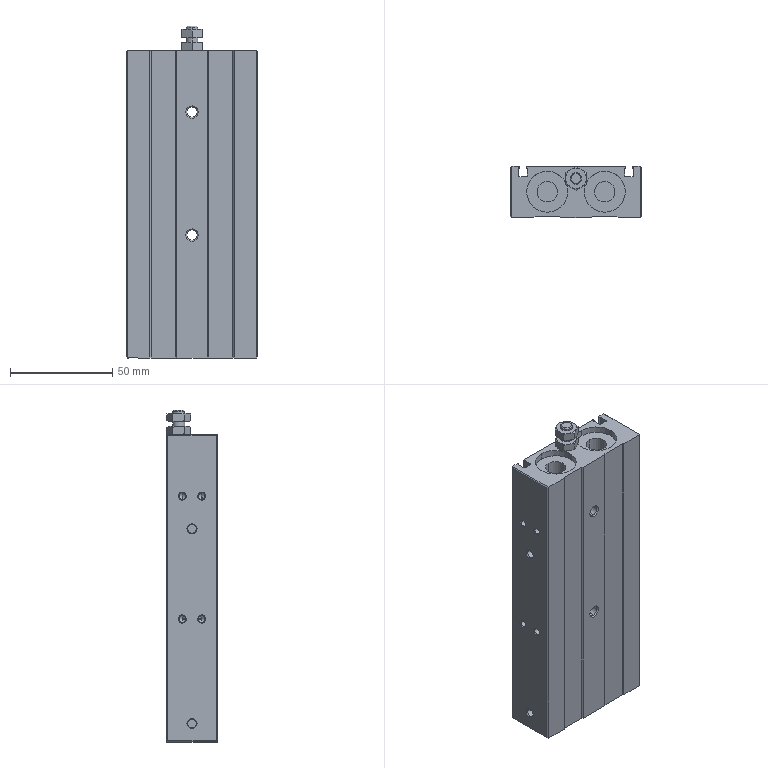Component | SolidWorks | TR-20x75-S-GN-1 (0)-3_TR-20x75-SCylinderBody-1 | 1 solid | 243 faces | volume 158415 mm3 | cylinder 94 | cone 77 | plane 72 | commonest cylinder face diameters 3.242 x16 4 x12 0.8 x12 20 x8 1.63 x8 4.134 x8 9.5 x4 21 x4